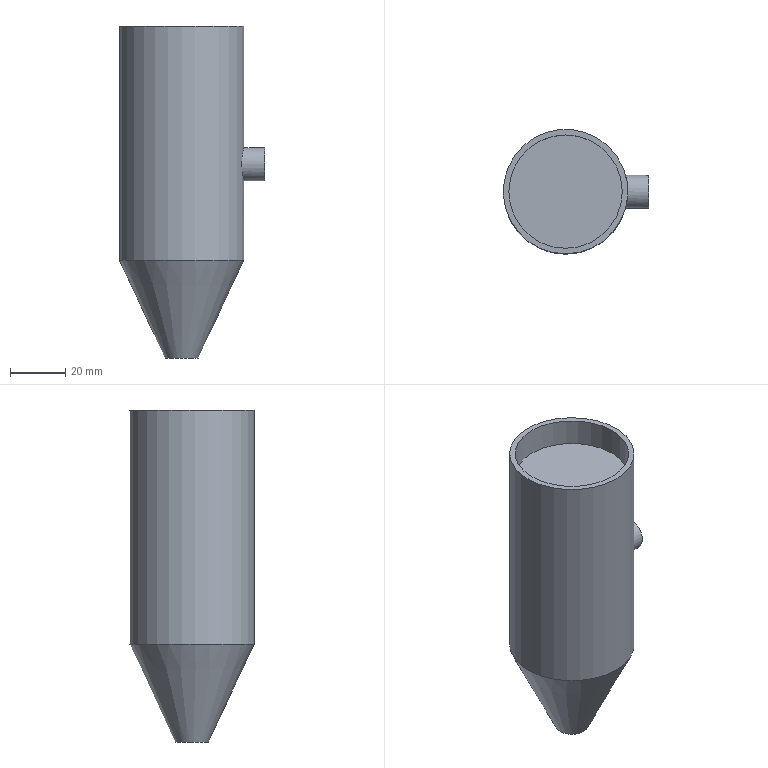Component | NX | GLUE_STICK | 1 solid | 8 faces | box 52.5 x 45 x 120 mm | volume 147340 mm3 | plane 4 | cylinder 3 | cone 1 | commonest cylinder face diameters 45 x1 41 x1 12 x1
STEP:
#1=CARTESIAN_POINT('',(0.,0.,0.));
#2=DIRECTION('',(0.,0.,1.));
#3=DIRECTION('',(1.,0.,0.));
#4=AXIS2_PLACEMENT_3D('',#1,#2,#3);
#5=CARTESIAN_POINT('',(674.689,-172.802,-1281.));
#6=VERTEX_POINT('',#5);
#7=CARTESIAN_POINT('',(674.689,-150.302,-1281.));
#8=DIRECTION('',(0.,0.,1.));
#9=DIRECTION('',(0.,-1.,0.));
#10=AXIS2_PLACEMENT_3D('',#7,#8,#9);
#11=CIRCLE('',#10,22.5);
#12=CARTESIAN_POINT('',(674.689,-150.302,-1225.));
#13=DIRECTION('',(0.,0.,1.));
#14=DIRECTION('',(0.,-1.,0.));
#15=AXIS2_PLACEMENT_3D('',#12,#13,#14);
#16=CYLINDRICAL_SURFACE('',#15,22.5);
#17=CARTESIAN_POINT('',(0.,-56.));
#18=DIRECTION('',(1.,0.));
#19=VECTOR('',#18,1.);
#20=LINE('',#17,#19);
#21=(GEOMETRIC_REPRESENTATION_CONTEXT(2)PARAMETRIC_REPRESENTATION_CONTEXT()REPRESENTATION_CONTEXT('',''));
#22=DEFINITIONAL_REPRESENTATION('',(#20),#21);
#23=PCURVE('',#16,#22);
#24=CARTESIAN_POINT('',(674.689,-172.802,-1281.));
#25=DIRECTION('',(0.,0.,-1.));
#26=DIRECTION('',(0.,1.,0.));
#27=AXIS2_PLACEMENT_3D('',#24,#25,#26);
#28=PLANE('',#27);
#29=CARTESIAN_POINT('',(0.,0.));
#30=CARTESIAN_POINT('',(0.,38.971));
#31=CARTESIAN_POINT('',(33.75,19.486));
#32=CARTESIAN_POINT('',(67.5,0.));
#33=CARTESIAN_POINT('',(33.75,-19.486));
#34=CARTESIAN_POINT('',(0.,-38.971));
#35=CARTESIAN_POINT('',(0.,0.));
#36=(BOUNDED_CURVE()B_SPLINE_CURVE(2,(#29,#30,#31,#32,#33,#34,#35),.UNSPECIFIED.,.T.,.F.)B_SPLINE_CURVE_WITH_KNOTS((1,2,2,2,2,1),(-2.094,0.,2.094,4.189,6.283,8.378),.UNSPECIFIED.)CURVE()GEOMETRIC_REPRESENTATION_ITEM()RATIONAL_B_SPLINE_CURVE((1.,0.5,1.,0.5,1.,0.5,1.))REPRESENTATION_ITEM(''));
#37=(GEOMETRIC_REPRESENTATION_CONTEXT(2)PARAMETRIC_REPRESENTATION_CONTEXT()REPRESENTATION_CONTEXT('',''));
#38=DEFINITIONAL_REPRESENTATION('',(#36),#37);
#39=PCURVE('',#28,#38);
#40=SURFACE_CURVE('',#11,(#23,#39),.PCURVE_S1.);
#41=EDGE_CURVE('',#6,#6,#40,.T.);
#42=ORIENTED_EDGE('',*,*,#41,.F.);
#43=CARTESIAN_POINT('',(674.689,-172.802,-1365.616));
#44=VERTEX_POINT('',#43);
#45=CARTESIAN_POINT('',(674.689,-172.802,-1365.616));
#46=CARTESIAN_POINT('',(674.689,-172.802,-1281.));
#47=B_SPLINE_CURVE_WITH_KNOTS('',1,(#45,#46),.UNSPECIFIED.,.F.,.F.,(2,2),(-140.616,-56.),.PIECEWISE_BEZIER_KNOTS.);
#48=CARTESIAN_POINT('',(0.,0.));
#49=DIRECTION('',(0.,1.));
#50=VECTOR('',#49,1.);
#51=LINE('',#48,#50);
#52=(GEOMETRIC_REPRESENTATION_CONTEXT(2)PARAMETRIC_REPRESENTATION_CONTEXT()REPRESENTATION_CONTEXT('',''));
#53=DEFINITIONAL_REPRESENTATION('',(#51),#52);
#54=PCURVE('',#16,#53);
#55=CARTESIAN_POINT('',(6.283,0.));
#56=DIRECTION('',(0.,1.));
#57=VECTOR('',#56,1.);
#58=LINE('',#55,#57);
#59=(GEOMETRIC_REPRESENTATION_CONTEXT(2)PARAMETRIC_REPRESENTATION_CONTEXT()REPRESENTATION_CONTEXT('',''));
#60=DEFINITIONAL_REPRESENTATION('',(#58),#59);
#61=PCURVE('',#16,#60);
#62=SEAM_CURVE('',#47,(#54,#61),.PCURVE_S1.);
#63=EDGE_CURVE('',#44,#6,#62,.T.);
#64=ORIENTED_EDGE('',*,*,#63,.F.);
#65=CARTESIAN_POINT('',(674.689,-150.302,-1365.616));
#66=DIRECTION('',(0.,0.,1.));
#67=DIRECTION('',(0.,-1.,0.));
#68=AXIS2_PLACEMENT_3D('',#65,#66,#67);
#69=CIRCLE('',#68,22.5);
#70=CARTESIAN_POINT('',(0.,-140.616));
#71=DIRECTION('',(1.,0.));
#72=VECTOR('',#71,1.);
#73=LINE('',#70,#72);
#74=(GEOMETRIC_REPRESENTATION_CONTEXT(2)PARAMETRIC_REPRESENTATION_CONTEXT()REPRESENTATION_CONTEXT('',''));
#75=DEFINITIONAL_REPRESENTATION('',(#73),#74);
#76=PCURVE('',#16,#75);
#77=CARTESIAN_POINT('',(674.689,-150.302,-1401.));
#78=DIRECTION('',(0.,0.,1.));
#79=DIRECTION('',(0.,-1.,0.));
#80=AXIS2_PLACEMENT_3D('',#77,#78,#79);
#81=CONICAL_SURFACE('',#80,6.,0.4363);
#82=CARTESIAN_POINT('',(0.,35.384));
#83=DIRECTION('',(1.,0.));
#84=VECTOR('',#83,1.);
#85=LINE('',#82,#84);
#86=(GEOMETRIC_REPRESENTATION_CONTEXT(2)PARAMETRIC_REPRESENTATION_CONTEXT()REPRESENTATION_CONTEXT('',''));
#87=DEFINITIONAL_REPRESENTATION('',(#85),#86);
#88=PCURVE('',#81,#87);
#89=SURFACE_CURVE('',#69,(#76,#88),.PCURVE_S1.);
#90=EDGE_CURVE('',#44,#44,#89,.T.);
#91=ORIENTED_EDGE('',*,*,#90,.T.);
#92=ORIENTED_EDGE('',*,*,#63,.T.);
#93=EDGE_LOOP('',(#42,#64,#91,#92));
#94=FACE_BOUND('',#93,.T.);
#95=CARTESIAN_POINT('',(696.374,-156.302,-1331.));
#96=VERTEX_POINT('',#95);
#97=CARTESIAN_POINT('',(696.374,-156.302,-1329.407));
#98=CARTESIAN_POINT('',(696.374,-156.302,-1332.593));
#99=CARTESIAN_POINT('',(696.574,-155.645,-1334.142));
#100=CARTESIAN_POINT('',(696.997,-153.442,-1336.344));
#101=CARTESIAN_POINT('',(697.189,-151.879,-1336.999));
#102=CARTESIAN_POINT('',(697.189,-148.732,-1337.001));
#103=CARTESIAN_POINT('',(696.999,-147.169,-1336.353));
#104=CARTESIAN_POINT('',(696.572,-144.949,-1334.132));
#105=CARTESIAN_POINT('',(696.374,-144.302,-1332.573));
#106=CARTESIAN_POINT('',(696.374,-144.301,-1329.432));
#107=CARTESIAN_POINT('',(696.572,-144.95,-1327.868));
#108=CARTESIAN_POINT('',(696.997,-147.162,-1325.653));
#109=CARTESIAN_POINT('',(697.189,-148.716,-1325.001));
#110=CARTESIAN_POINT('',(697.189,-151.882,-1324.999));
#111=CARTESIAN_POINT('',(696.997,-153.441,-1325.655));
#112=CARTESIAN_POINT('',(696.574,-155.644,-1327.855));
#113=CARTESIAN_POINT('',(696.374,-156.302,-1329.407));
#114=CARTESIAN_POINT('',(696.374,-156.302,-1332.593));
#115=B_SPLINE_CURVE_WITH_KNOTS('',3,(#97,#98,#99,#100,#101,#102,#103,#104,#105,#106,#107,#108,#109,#110,#111,#112,#113,#114),.UNSPECIFIED.,.T.,.F.,(2,2,2,2,2,2,2,2,2,2,2),(-0.125,0.,0.125,0.25,0.375,0.5,0.625,0.75,0.875,1.,1.125),.UNSPECIFIED.);
#116=CARTESIAN_POINT('',(1.301,-106.));
#117=CARTESIAN_POINT('',(1.301,-106.29));
#118=CARTESIAN_POINT('',(1.303,-106.866));
#119=CARTESIAN_POINT('',(1.312,-107.707));
#120=CARTESIAN_POINT('',(1.325,-108.511));
#121=CARTESIAN_POINT('',(1.344,-109.262));
#122=CARTESIAN_POINT('',(1.367,-109.946));
#123=CARTESIAN_POINT('',(1.395,-110.548));
#124=CARTESIAN_POINT('',(1.425,-111.057));
#125=CARTESIAN_POINT('',(1.459,-111.466));
#126=CARTESIAN_POINT('',(1.495,-111.769));
#127=CARTESIAN_POINT('',(1.533,-111.956));
#128=CARTESIAN_POINT('',(1.571,-112.022));
#129=CARTESIAN_POINT('',(1.609,-111.958));
#130=CARTESIAN_POINT('',(1.646,-111.772));
#131=CARTESIAN_POINT('',(1.682,-111.471));
#132=CARTESIAN_POINT('',(1.716,-111.061));
#133=CARTESIAN_POINT('',(1.747,-110.55));
#134=CARTESIAN_POINT('',(1.774,-109.942));
#135=CARTESIAN_POINT('',(1.798,-109.254));
#136=CARTESIAN_POINT('',(1.816,-108.5));
#137=CARTESIAN_POINT('',(1.83,-107.696));
#138=CARTESIAN_POINT('',(1.839,-106.859));
#139=CARTESIAN_POINT('',(1.842,-106.003));
#140=CARTESIAN_POINT('',(1.839,-105.146));
#141=CARTESIAN_POINT('',(1.83,-104.308));
#142=CARTESIAN_POINT('',(1.816,-103.503));
#143=CARTESIAN_POINT('',(1.798,-102.748));
#144=CARTESIAN_POINT('',(1.774,-102.06));
#145=CARTESIAN_POINT('',(1.747,-101.454));
#146=CARTESIAN_POINT('',(1.716,-100.943));
#147=CARTESIAN_POINT('',(1.682,-100.533));
#148=CARTESIAN_POINT('',(1.647,-100.231));
#149=CARTESIAN_POINT('',(1.609,-100.043));
#150=CARTESIAN_POINT('',(1.571,-99.978));
#151=CARTESIAN_POINT('',(1.533,-100.043));
#152=CARTESIAN_POINT('',(1.495,-100.23));
#153=CARTESIAN_POINT('',(1.459,-100.532));
#154=CARTESIAN_POINT('',(1.426,-100.942));
#155=CARTESIAN_POINT('',(1.395,-101.451));
#156=CARTESIAN_POINT('',(1.367,-102.052));
#157=CARTESIAN_POINT('',(1.344,-102.737));
#158=CARTESIAN_POINT('',(1.325,-103.488));
#159=CARTESIAN_POINT('',(1.312,-104.292));
#160=CARTESIAN_POINT('',(1.303,-105.134));
#161=CARTESIAN_POINT('',(1.301,-105.71));
#162=CARTESIAN_POINT('',(1.301,-106.));
#163=B_SPLINE_CURVE_WITH_KNOTS('',3,(#116,#117,#118,#119,#120,#121,#122,#123,#124,#125,#126,#127,#128,#129,#130,#131,#132,#133,#134,#135,#136,#137,#138,#139,#140,#141,#142,#143,#144,#145,#146,#147,#148,#149,#150,#151,#152,#153,#154,#155,#156,#157,#158,#159,#160,#161,#162),.UNSPECIFIED.,.T.,.F.,(4,1,1,1,1,1,1,1,1,1,1,1,1,1,1,1,1,1,1,1,1,1,1,1,1,1,1,1,1,1,1,1,1,1,1,1,1,1,1,1,1,1,1,1,4),(0.,0.02273,0.04545,0.06818,0.09091,0.1136,0.1364,0.1591,0.1818,0.2045,0.2273,0.25,0.2727,0.2955,0.3182,0.3409,0.3636,0.3864,0.4091,0.4318,0.4545,0.4773,0.5,0.5227,0.5455,0.5682,0.5909,0.6136,0.6364,0.6591,0.6818,0.7045,0.7273,0.75,0.7727,0.7955,0.8182,0.8409,0.8636,0.8864,0.9091,0.9318,0.9545,0.9773,1.),.QUASI_UNIFORM_KNOTS.);
#164=(GEOMETRIC_REPRESENTATION_CONTEXT(2)PARAMETRIC_REPRESENTATION_CONTEXT()REPRESENTATION_CONTEXT('',''));
#165=DEFINITIONAL_REPRESENTATION('',(#163),#164);
#166=PCURVE('',#16,#165);
#167=CARTESIAN_POINT('',(704.689,-150.302,-1331.));
#168=DIRECTION('',(-1.,0.,0.));
#169=DIRECTION('',(0.,-1.,0.));
#170=AXIS2_PLACEMENT_3D('',#167,#168,#169);
#171=CYLINDRICAL_SURFACE('',#170,6.);
#172=CARTESIAN_POINT('',(6.283,8.315));
#173=CARTESIAN_POINT('',(6.235,8.315));
#174=CARTESIAN_POINT('',(6.139,8.302));
#175=CARTESIAN_POINT('',(5.995,8.249));
#176=CARTESIAN_POINT('',(5.853,8.17));
#177=CARTESIAN_POINT('',(5.71,8.072));
#178=CARTESIAN_POINT('',(5.568,7.962));
#179=CARTESIAN_POINT('',(5.427,7.845));
#180=CARTESIAN_POINT('',(5.285,7.736));
#181=CARTESIAN_POINT('',(5.142,7.64));
#182=CARTESIAN_POINT('',(4.999,7.564));
#183=CARTESIAN_POINT('',(4.856,7.513));
#184=CARTESIAN_POINT('',(4.713,7.494));
#185=CARTESIAN_POINT('',(4.57,7.512));
#186=CARTESIAN_POINT('',(4.427,7.563));
#187=CARTESIAN_POINT('',(4.284,7.639));
#188=CARTESIAN_POINT('',(4.141,7.735));
#189=CARTESIAN_POINT('',(3.998,7.845));
#190=CARTESIAN_POINT('',(3.856,7.962));
#191=CARTESIAN_POINT('',(3.713,8.073));
#192=CARTESIAN_POINT('',(3.57,8.171));
#193=CARTESIAN_POINT('',(3.427,8.249));
#194=CARTESIAN_POINT('',(3.285,8.302));
#195=CARTESIAN_POINT('',(3.142,8.321));
#196=CARTESIAN_POINT('',(2.999,8.302));
#197=CARTESIAN_POINT('',(2.856,8.249));
#198=CARTESIAN_POINT('',(2.713,8.171));
#199=CARTESIAN_POINT('',(2.571,8.073));
#200=CARTESIAN_POINT('',(2.428,7.963));
#201=CARTESIAN_POINT('',(2.286,7.846));
#202=CARTESIAN_POINT('',(2.143,7.736));
#203=CARTESIAN_POINT('',(2.001,7.64));
#204=CARTESIAN_POINT('',(1.858,7.564));
#205=CARTESIAN_POINT('',(1.715,7.513));
#206=CARTESIAN_POINT('',(1.571,7.494));
#207=CARTESIAN_POINT('',(1.428,7.513));
#208=CARTESIAN_POINT('',(1.284,7.563));
#209=CARTESIAN_POINT('',(1.141,7.64));
#210=CARTESIAN_POINT('',(0.9987,7.736));
#211=CARTESIAN_POINT('',(0.8566,7.845));
#212=CARTESIAN_POINT('',(0.7152,7.961));
#213=CARTESIAN_POINT('',(0.5733,8.072));
#214=CARTESIAN_POINT('',(0.4309,8.17));
#215=CARTESIAN_POINT('',(0.2879,8.249));
#216=CARTESIAN_POINT('',(0.1444,8.302));
#217=CARTESIAN_POINT('',(0.04825,8.315));
#218=CARTESIAN_POINT('',(0.,8.315));
#219=B_SPLINE_CURVE_WITH_KNOTS('',3,(#172,#173,#174,#175,#176,#177,#178,#179,#180,#181,#182,#183,#184,#185,#186,#187,#188,#189,#190,#191,#192,#193,#194,#195,#196,#197,#198,#199,#200,#201,#202,#203,#204,#205,#206,#207,#208,#209,#210,#211,#212,#213,#214,#215,#216,#217,#218),.UNSPECIFIED.,.F.,.F.,(4,1,1,1,1,1,1,1,1,1,1,1,1,1,1,1,1,1,1,1,1,1,1,1,1,1,1,1,1,1,1,1,1,1,1,1,1,1,1,1,1,1,1,1,4),(0.,0.02273,0.04545,0.06818,0.09091,0.1136,0.1364,0.1591,0.1818,0.2045,0.2273,0.25,0.2727,0.2955,0.3182,0.3409,0.3636,0.3864,0.4091,0.4318,0.4545,0.4773,0.5,0.5227,0.5455,0.5682,0.5909,0.6136,0.6364,0.6591,0.6818,0.7045,0.7273,0.75,0.7727,0.7955,0.8182,0.8409,0.8636,0.8864,0.9091,0.9318,0.9545,0.9773,1.),.QUASI_UNIFORM_KNOTS.);
#220=(GEOMETRIC_REPRESENTATION_CONTEXT(2)PARAMETRIC_REPRESENTATION_CONTEXT()REPRESENTATION_CONTEXT('',''));
#221=DEFINITIONAL_REPRESENTATION('',(#219),#220);
#222=PCURVE('',#171,#221);
#223=SURFACE_CURVE('',#115,(#166,#222),.PCURVE_S1.);
#224=EDGE_CURVE('',#96,#96,#223,.T.);
#225=ORIENTED_EDGE('',*,*,#224,.F.);
#226=EDGE_LOOP('',(#225));
#227=FACE_BOUND('',#226,.T.);
#228=ADVANCED_FACE('',(#94,#227),#16,.T.);
#229=CARTESIAN_POINT('',(674.689,-156.302,-1401.));
#230=VERTEX_POINT('',#229);
#231=CARTESIAN_POINT('',(674.689,-150.302,-1401.));
#232=DIRECTION('',(0.,0.,1.));
#233=DIRECTION('',(0.,-1.,0.));
#234=AXIS2_PLACEMENT_3D('',#231,#232,#233);
#235=CIRCLE('',#234,6.);
#236=CARTESIAN_POINT('',(674.689,-150.302,-1401.));
#237=DIRECTION('',(0.,0.,1.));
#238=DIRECTION('',(0.,-1.,0.));
#239=AXIS2_PLACEMENT_3D('',#236,#237,#238);
#240=PLANE('',#239);
#241=CARTESIAN_POINT('',(0.,0.));
#242=DIRECTION('',(1.,0.));
#243=AXIS2_PLACEMENT_2D('',#241,#242);
#244=CIRCLE('',#243,6.);
#245=(GEOMETRIC_REPRESENTATION_CONTEXT(2)PARAMETRIC_REPRESENTATION_CONTEXT()REPRESENTATION_CONTEXT('',''));
#246=DEFINITIONAL_REPRESENTATION('',(#244),#245);
#247=PCURVE('',#240,#246);
#248=CARTESIAN_POINT('',(0.,0.));
#249=DIRECTION('',(1.,0.));
#250=VECTOR('',#249,1.);
#251=LINE('',#248,#250);
#252=(GEOMETRIC_REPRESENTATION_CONTEXT(2)PARAMETRIC_REPRESENTATION_CONTEXT()REPRESENTATION_CONTEXT('',''));
#253=DEFINITIONAL_REPRESENTATION('',(#251),#252);
#254=PCURVE('',#81,#253);
#255=SURFACE_CURVE('',#235,(#247,#254),.PCURVE_S1.);
#256=EDGE_CURVE('',#230,#230,#255,.T.);
#257=ORIENTED_EDGE('',*,*,#256,.F.);
#258=EDGE_LOOP('',(#257));
#259=FACE_BOUND('',#258,.T.);
#260=ADVANCED_FACE('',(#259),#240,.F.);
#261=CARTESIAN_POINT('',(674.689,-170.802,-1291.));
#262=VERTEX_POINT('',#261);
#263=CARTESIAN_POINT('',(674.689,-150.302,-1291.));
#264=DIRECTION('',(0.,0.,1.));
#265=DIRECTION('',(0.,-1.,0.));
#266=AXIS2_PLACEMENT_3D('',#263,#264,#265);
#267=CIRCLE('',#266,20.5);
#268=CARTESIAN_POINT('',(674.689,-170.802,-1291.));
#269=DIRECTION('',(0.,0.,-1.));
#270=DIRECTION('',(0.,1.,0.));
#271=AXIS2_PLACEMENT_3D('',#268,#269,#270);
#272=PLANE('',#271);
#273=CARTESIAN_POINT('',(0.,0.));
#274=CARTESIAN_POINT('',(0.,35.507));
#275=CARTESIAN_POINT('',(30.75,17.754));
#276=CARTESIAN_POINT('',(61.5,0.));
#277=CARTESIAN_POINT('',(30.75,-17.754));
#278=CARTESIAN_POINT('',(0.,-35.507));
#279=CARTESIAN_POINT('',(0.,0.));
#280=(BOUNDED_CURVE()B_SPLINE_CURVE(2,(#273,#274,#275,#276,#277,#278,#279),.UNSPECIFIED.,.T.,.F.)B_SPLINE_CURVE_WITH_KNOTS((1,2,2,2,2,1),(-2.094,0.,2.094,4.189,6.283,8.378),.UNSPECIFIED.)CURVE()GEOMETRIC_REPRESENTATION_ITEM()RATIONAL_B_SPLINE_CURVE((1.,0.5,1.,0.5,1.,0.5,1.))REPRESENTATION_ITEM(''));
#281=(GEOMETRIC_REPRESENTATION_CONTEXT(2)PARAMETRIC_REPRESENTATION_CONTEXT()REPRESENTATION_CONTEXT('',''));
#282=DEFINITIONAL_REPRESENTATION('',(#280),#281);
#283=PCURVE('',#272,#282);
#284=CARTESIAN_POINT('',(674.689,-150.302,-1225.));
#285=DIRECTION('',(0.,0.,1.));
#286=DIRECTION('',(0.,-1.,0.));
#287=AXIS2_PLACEMENT_3D('',#284,#285,#286);
#288=CYLINDRICAL_SURFACE('',#287,20.5);
#289=CARTESIAN_POINT('',(0.,-66.));
#290=DIRECTION('',(1.,0.));
#291=VECTOR('',#290,1.);
#292=LINE('',#289,#291);
#293=(GEOMETRIC_REPRESENTATION_CONTEXT(2)PARAMETRIC_REPRESENTATION_CONTEXT()REPRESENTATION_CONTEXT('',''));
#294=DEFINITIONAL_REPRESENTATION('',(#292),#293);
#295=PCURVE('',#288,#294);
#296=SURFACE_CURVE('',#267,(#283,#295),.PCURVE_S1.);
#297=EDGE_CURVE('',#262,#262,#296,.T.);
#298=ORIENTED_EDGE('',*,*,#297,.T.);
#299=EDGE_LOOP('',(#298));
#300=FACE_BOUND('',#299,.T.);
#301=ADVANCED_FACE('',(#300),#272,.F.);
#302=ORIENTED_EDGE('',*,*,#297,.T.);
#303=CARTESIAN_POINT('',(674.689,-170.802,-1281.));
#304=VERTEX_POINT('',#303);
#305=CARTESIAN_POINT('',(674.689,-170.802,-1291.));
#306=CARTESIAN_POINT('',(674.689,-170.802,-1281.));
#307=B_SPLINE_CURVE_WITH_KNOTS('',1,(#305,#306),.UNSPECIFIED.,.F.,.F.,(2,2),(-66.,-56.),.PIECEWISE_BEZIER_KNOTS.);
#308=CARTESIAN_POINT('',(6.283,0.));
#309=DIRECTION('',(0.,1.));
#310=VECTOR('',#309,1.);
#311=LINE('',#308,#310);
#312=(GEOMETRIC_REPRESENTATION_CONTEXT(2)PARAMETRIC_REPRESENTATION_CONTEXT()REPRESENTATION_CONTEXT('',''));
#313=DEFINITIONAL_REPRESENTATION('',(#311),#312);
#314=PCURVE('',#288,#313);
#315=CARTESIAN_POINT('',(0.,0.));
#316=DIRECTION('',(0.,1.));
#317=VECTOR('',#316,1.);
#318=LINE('',#315,#317);
#319=(GEOMETRIC_REPRESENTATION_CONTEXT(2)PARAMETRIC_REPRESENTATION_CONTEXT()REPRESENTATION_CONTEXT('',''));
#320=DEFINITIONAL_REPRESENTATION('',(#318),#319);
#321=PCURVE('',#288,#320);
#322=SEAM_CURVE('',#307,(#314,#321),.PCURVE_S1.);
#323=EDGE_CURVE('',#262,#304,#322,.T.);
#324=ORIENTED_EDGE('',*,*,#323,.T.);
#325=CARTESIAN_POINT('',(674.689,-150.302,-1281.));
#326=DIRECTION('',(0.,0.,1.));
#327=DIRECTION('',(0.,-1.,0.));
#328=AXIS2_PLACEMENT_3D('',#325,#326,#327);
#329=CIRCLE('',#328,20.5);
#330=CARTESIAN_POINT('',(0.,-56.));
#331=DIRECTION('',(1.,0.));
#332=VECTOR('',#331,1.);
#333=LINE('',#330,#332);
#334=(GEOMETRIC_REPRESENTATION_CONTEXT(2)PARAMETRIC_REPRESENTATION_CONTEXT()REPRESENTATION_CONTEXT('',''));
#335=DEFINITIONAL_REPRESENTATION('',(#333),#334);
#336=PCURVE('',#288,#335);
#337=CARTESIAN_POINT('',(2.,0.));
#338=CARTESIAN_POINT('',(2.,35.507));
#339=CARTESIAN_POINT('',(32.75,17.754));
#340=CARTESIAN_POINT('',(63.5,0.));
#341=CARTESIAN_POINT('',(32.75,-17.754));
#342=CARTESIAN_POINT('',(2.,-35.507));
#343=CARTESIAN_POINT('',(2.,0.));
#344=(BOUNDED_CURVE()B_SPLINE_CURVE(2,(#337,#338,#339,#340,#341,#342,#343),.UNSPECIFIED.,.T.,.F.)B_SPLINE_CURVE_WITH_KNOTS((1,2,2,2,2,1),(-2.094,0.,2.094,4.189,6.283,8.378),.UNSPECIFIED.)CURVE()GEOMETRIC_REPRESENTATION_ITEM()RATIONAL_B_SPLINE_CURVE((1.,0.5,1.,0.5,1.,0.5,1.))REPRESENTATION_ITEM(''));
#345=(GEOMETRIC_REPRESENTATION_CONTEXT(2)PARAMETRIC_REPRESENTATION_CONTEXT()REPRESENTATION_CONTEXT('',''));
#346=DEFINITIONAL_REPRESENTATION('',(#344),#345);
#347=PCURVE('',#28,#346);
#348=SURFACE_CURVE('',#329,(#336,#347),.PCURVE_S1.);
#349=EDGE_CURVE('',#304,#304,#348,.T.);
#350=ORIENTED_EDGE('',*,*,#349,.F.);
#351=ORIENTED_EDGE('',*,*,#323,.F.);
#352=EDGE_LOOP('',(#302,#324,#350,#351));
#353=FACE_BOUND('',#352,.F.);
#354=ADVANCED_FACE('',(#353),#288,.F.);
#355=ORIENTED_EDGE('',*,*,#349,.F.);
#356=EDGE_LOOP('',(#355));
#357=FACE_BOUND('',#356,.T.);
#358=ORIENTED_EDGE('',*,*,#41,.T.);
#359=EDGE_LOOP('',(#358));
#360=FACE_BOUND('',#359,.T.);
#361=ADVANCED_FACE('',(#357,#360),#28,.F.);
#362=ORIENTED_EDGE('',*,*,#90,.F.);
#363=CARTESIAN_POINT('',(674.689,-156.302,-1401.));
#364=CARTESIAN_POINT('',(674.689,-172.802,-1365.616));
#365=B_SPLINE_CURVE_WITH_KNOTS('',1,(#363,#364),.UNSPECIFIED.,.F.,.F.,(2,2),(0.,39.042),.PIECEWISE_BEZIER_KNOTS.);
#366=CARTESIAN_POINT('',(0.,0.));
#367=DIRECTION('',(0.,1.));
#368=VECTOR('',#367,1.);
#369=LINE('',#366,#368);
#370=(GEOMETRIC_REPRESENTATION_CONTEXT(2)PARAMETRIC_REPRESENTATION_CONTEXT()REPRESENTATION_CONTEXT('',''));
#371=DEFINITIONAL_REPRESENTATION('',(#369),#370);
#372=PCURVE('',#81,#371);
#373=CARTESIAN_POINT('',(6.283,0.));
#374=DIRECTION('',(0.,1.));
#375=VECTOR('',#374,1.);
#376=LINE('',#373,#375);
#377=(GEOMETRIC_REPRESENTATION_CONTEXT(2)PARAMETRIC_REPRESENTATION_CONTEXT()REPRESENTATION_CONTEXT('',''));
#378=DEFINITIONAL_REPRESENTATION('',(#376),#377);
#379=PCURVE('',#81,#378);
#380=SEAM_CURVE('',#365,(#372,#379),.PCURVE_S1.);
#381=EDGE_CURVE('',#230,#44,#380,.T.);
#382=ORIENTED_EDGE('',*,*,#381,.F.);
#383=ORIENTED_EDGE('',*,*,#256,.T.);
#384=ORIENTED_EDGE('',*,*,#381,.T.);
#385=EDGE_LOOP('',(#362,#382,#383,#384));
#386=FACE_BOUND('',#385,.T.);
#387=ADVANCED_FACE('',(#386),#81,.T.);
#388=CARTESIAN_POINT('',(704.689,-156.302,-1331.));
#389=VERTEX_POINT('',#388);
#390=CARTESIAN_POINT('',(704.689,-150.302,-1325.));
#391=VERTEX_POINT('',#390);
#392=CARTESIAN_POINT('',(704.689,-150.302,-1331.));
#393=DIRECTION('',(1.,0.,0.));
#394=DIRECTION('',(0.,0.,1.));
#395=AXIS2_PLACEMENT_3D('',#392,#393,#394);
#396=CIRCLE('',#395,6.);
#397=CARTESIAN_POINT('',(7.854,0.));
#398=DIRECTION('',(-1.,0.));
#399=VECTOR('',#398,1.);
#400=LINE('',#397,#399);
#401=(GEOMETRIC_REPRESENTATION_CONTEXT(2)PARAMETRIC_REPRESENTATION_CONTEXT()REPRESENTATION_CONTEXT('',''));
#402=DEFINITIONAL_REPRESENTATION('',(#400),#401);
#403=PCURVE('',#171,#402);
#404=CARTESIAN_POINT('',(704.689,-150.302,-1331.));
#405=DIRECTION('',(1.,0.,0.));
#406=DIRECTION('',(0.,1.,0.));
#407=AXIS2_PLACEMENT_3D('',#404,#405,#406);
#408=PLANE('',#407);
#409=CARTESIAN_POINT('',(0.,0.));
#410=DIRECTION('',(0.,1.));
#411=AXIS2_PLACEMENT_2D('',#409,#410);
#412=CIRCLE('',#411,6.);
#413=(GEOMETRIC_REPRESENTATION_CONTEXT(2)PARAMETRIC_REPRESENTATION_CONTEXT()REPRESENTATION_CONTEXT('',''));
#414=DEFINITIONAL_REPRESENTATION('',(#412),#413);
#415=PCURVE('',#408,#414);
#416=SURFACE_CURVE('',#396,(#403,#415),.PCURVE_S1.);
#417=EDGE_CURVE('',#389,#391,#416,.T.);
#418=ORIENTED_EDGE('',*,*,#417,.F.);
#419=CARTESIAN_POINT('',(704.689,-156.302,-1331.));
#420=CARTESIAN_POINT('',(696.374,-156.302,-1331.));
#421=B_SPLINE_CURVE_WITH_KNOTS('',1,(#419,#420),.UNSPECIFIED.,.F.,.F.,(2,2),(0.,8.315),.PIECEWISE_BEZIER_KNOTS.);
#422=CARTESIAN_POINT('',(6.283,0.));
#423=DIRECTION('',(0.,1.));
#424=VECTOR('',#423,1.);
#425=LINE('',#422,#424);
#426=(GEOMETRIC_REPRESENTATION_CONTEXT(2)PARAMETRIC_REPRESENTATION_CONTEXT()REPRESENTATION_CONTEXT('',''));
#427=DEFINITIONAL_REPRESENTATION('',(#425),#426);
#428=PCURVE('',#171,#427);
#429=CARTESIAN_POINT('',(0.,0.));
#430=DIRECTION('',(0.,1.));
#431=VECTOR('',#430,1.);
#432=LINE('',#429,#431);
#433=(GEOMETRIC_REPRESENTATION_CONTEXT(2)PARAMETRIC_REPRESENTATION_CONTEXT()REPRESENTATION_CONTEXT('',''));
#434=DEFINITIONAL_REPRESENTATION('',(#432),#433);
#435=PCURVE('',#171,#434);
#436=SEAM_CURVE('',#421,(#428,#435),.PCURVE_S1.);
#437=EDGE_CURVE('',#389,#96,#436,.T.);
#438=ORIENTED_EDGE('',*,*,#437,.T.);
#439=ORIENTED_EDGE('',*,*,#224,.T.);
#440=ORIENTED_EDGE('',*,*,#437,.F.);
#441=CARTESIAN_POINT('',(704.689,-150.302,-1331.));
#442=DIRECTION('',(1.,0.,0.));
#443=DIRECTION('',(0.,0.,1.));
#444=AXIS2_PLACEMENT_3D('',#441,#442,#443);
#445=CIRCLE('',#444,6.);
#446=CARTESIAN_POINT('',(1.571,0.));
#447=DIRECTION('',(-1.,0.));
#448=VECTOR('',#447,1.);
#449=LINE('',#446,#448);
#450=(GEOMETRIC_REPRESENTATION_CONTEXT(2)PARAMETRIC_REPRESENTATION_CONTEXT()REPRESENTATION_CONTEXT('',''));
#451=DEFINITIONAL_REPRESENTATION('',(#449),#450);
#452=PCURVE('',#171,#451);
#453=CARTESIAN_POINT('',(0.,0.));
#454=DIRECTION('',(0.,1.));
#455=AXIS2_PLACEMENT_2D('',#453,#454);
#456=CIRCLE('',#455,6.);
#457=(GEOMETRIC_REPRESENTATION_CONTEXT(2)PARAMETRIC_REPRESENTATION_CONTEXT()REPRESENTATION_CONTEXT('',''));
#458=DEFINITIONAL_REPRESENTATION('',(#456),#457);
#459=PCURVE('',#408,#458);
#460=SURFACE_CURVE('',#445,(#452,#459),.PCURVE_S1.);
#461=EDGE_CURVE('',#391,#389,#460,.T.);
#462=ORIENTED_EDGE('',*,*,#461,.F.);
#463=EDGE_LOOP('',(#418,#438,#439,#440,#462));
#464=FACE_BOUND('',#463,.T.);
#465=ADVANCED_FACE('',(#464),#171,.T.);
#466=ORIENTED_EDGE('',*,*,#461,.T.);
#467=ORIENTED_EDGE('',*,*,#417,.T.);
#468=EDGE_LOOP('',(#466,#467));
#469=FACE_BOUND('',#468,.T.);
#470=ADVANCED_FACE('',(#469),#408,.T.);
#471=CLOSED_SHELL('',(#228,#260,#301,#354,#361,#387,#465,#470));
#472=MANIFOLD_SOLID_BREP('',#471);
#473=(LENGTH_UNIT()NAMED_UNIT(*)SI_UNIT(.MILLI.,.METRE.));
#474=UNCERTAINTY_MEASURE_WITH_UNIT(LENGTH_MEASURE(0.001),#473,'','');
#475=(NAMED_UNIT(*)PLANE_ANGLE_UNIT()SI_UNIT($,.RADIAN.));
#476=(NAMED_UNIT(*)SI_UNIT($,.STERADIAN.)SOLID_ANGLE_UNIT());
#477=(GEOMETRIC_REPRESENTATION_CONTEXT(3)GLOBAL_UNCERTAINTY_ASSIGNED_CONTEXT((#474))GLOBAL_UNIT_ASSIGNED_CONTEXT((#473,#475,#476))REPRESENTATION_CONTEXT('',''));
#478=ADVANCED_BREP_SHAPE_REPRESENTATION('',(#4,#472),#477);